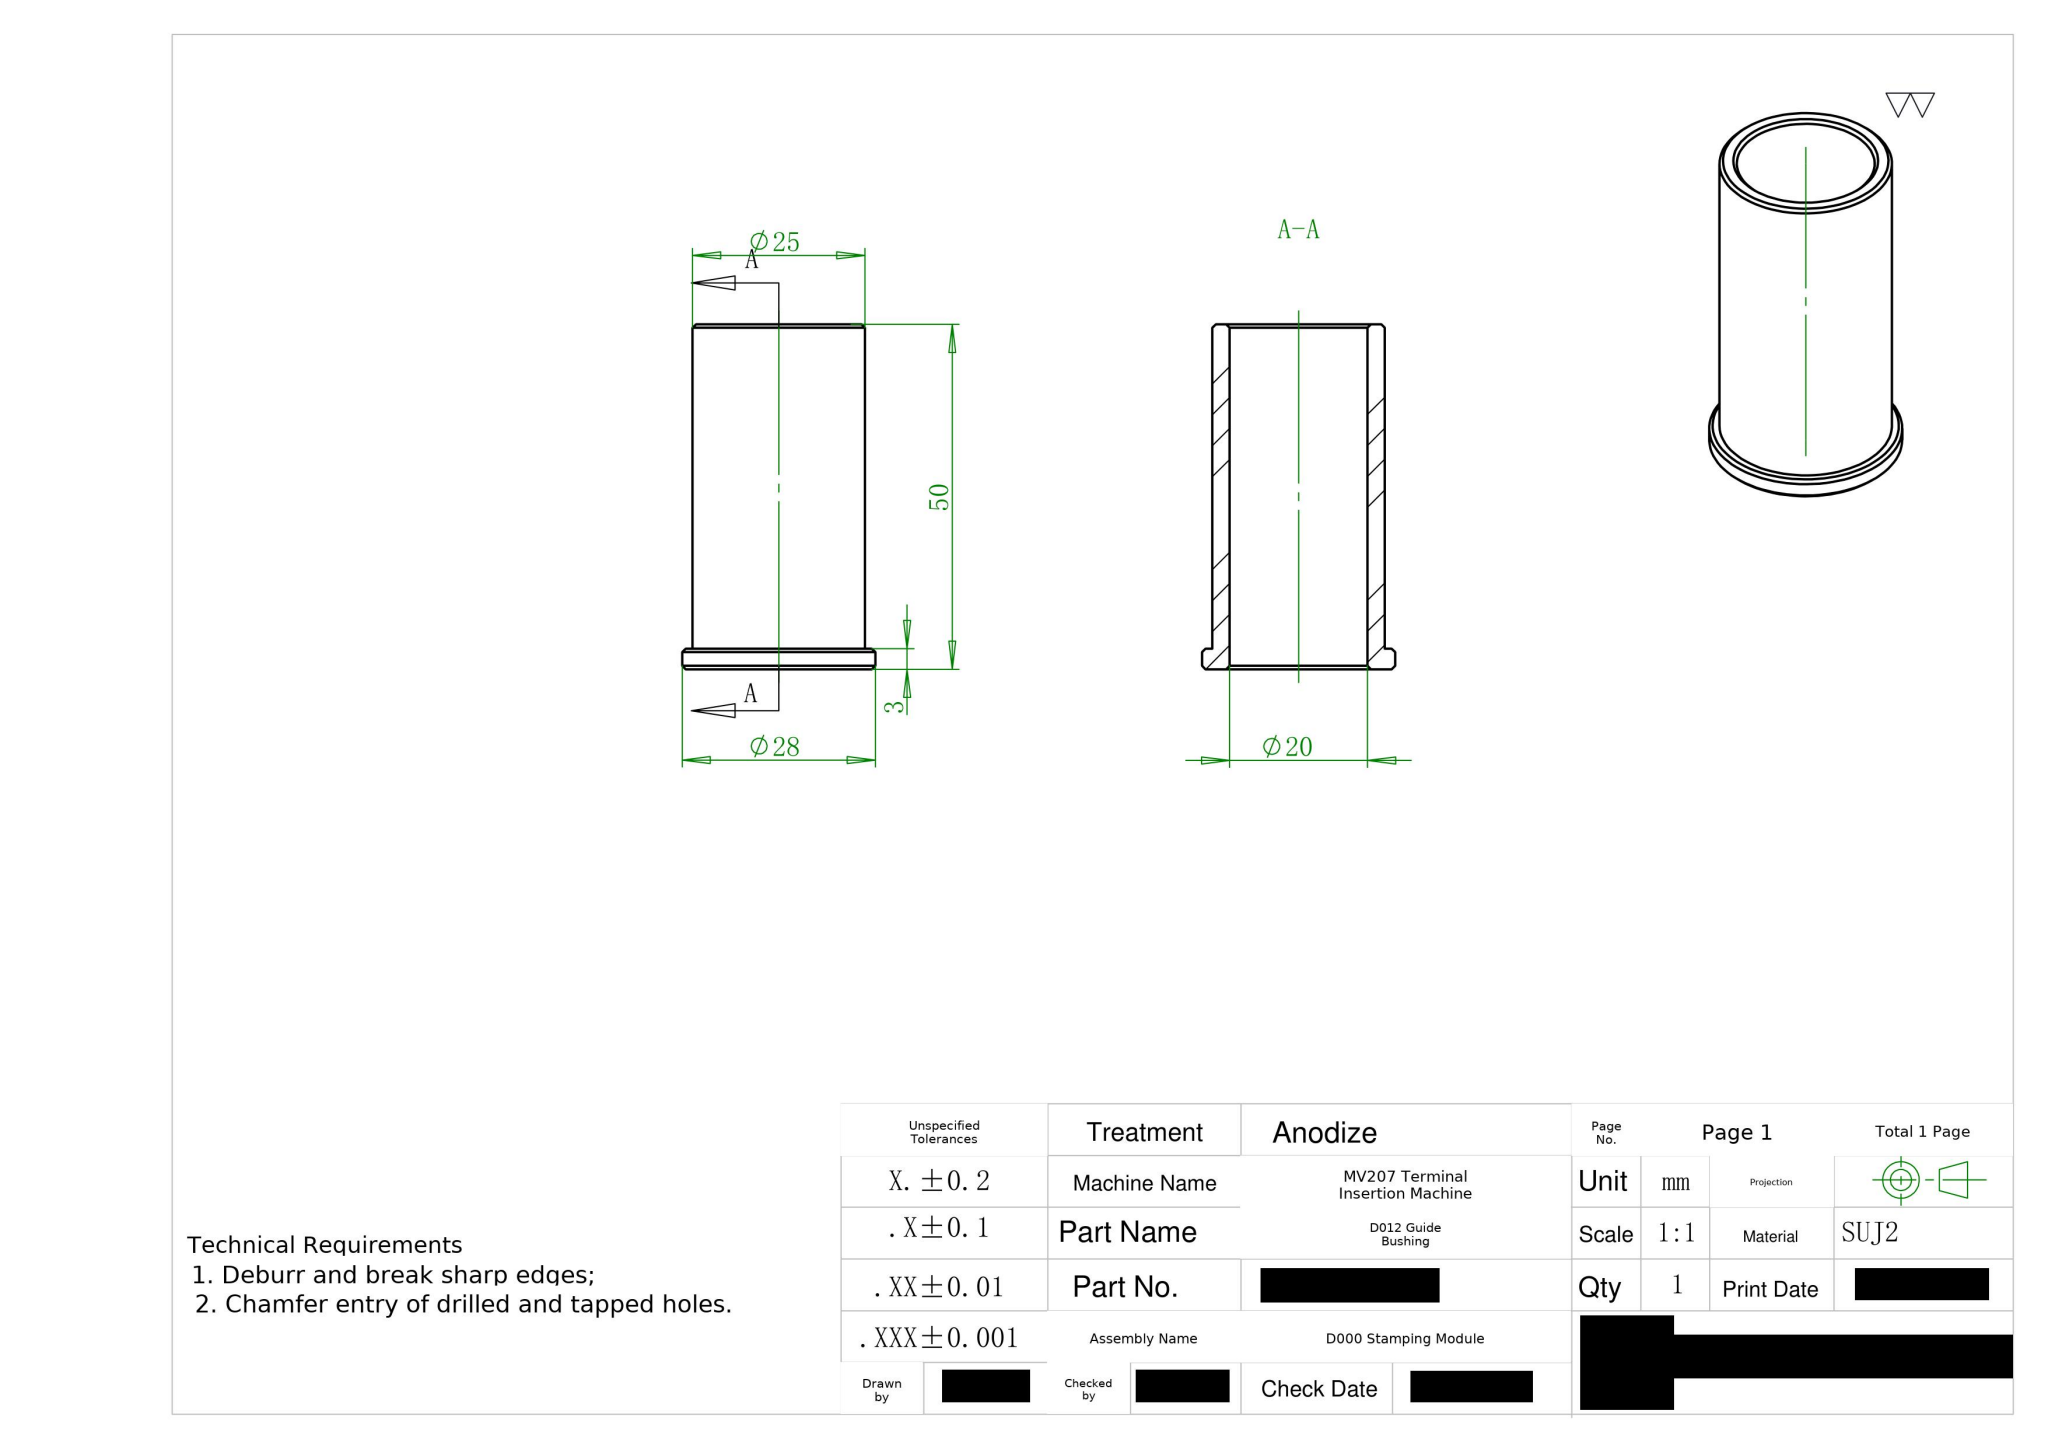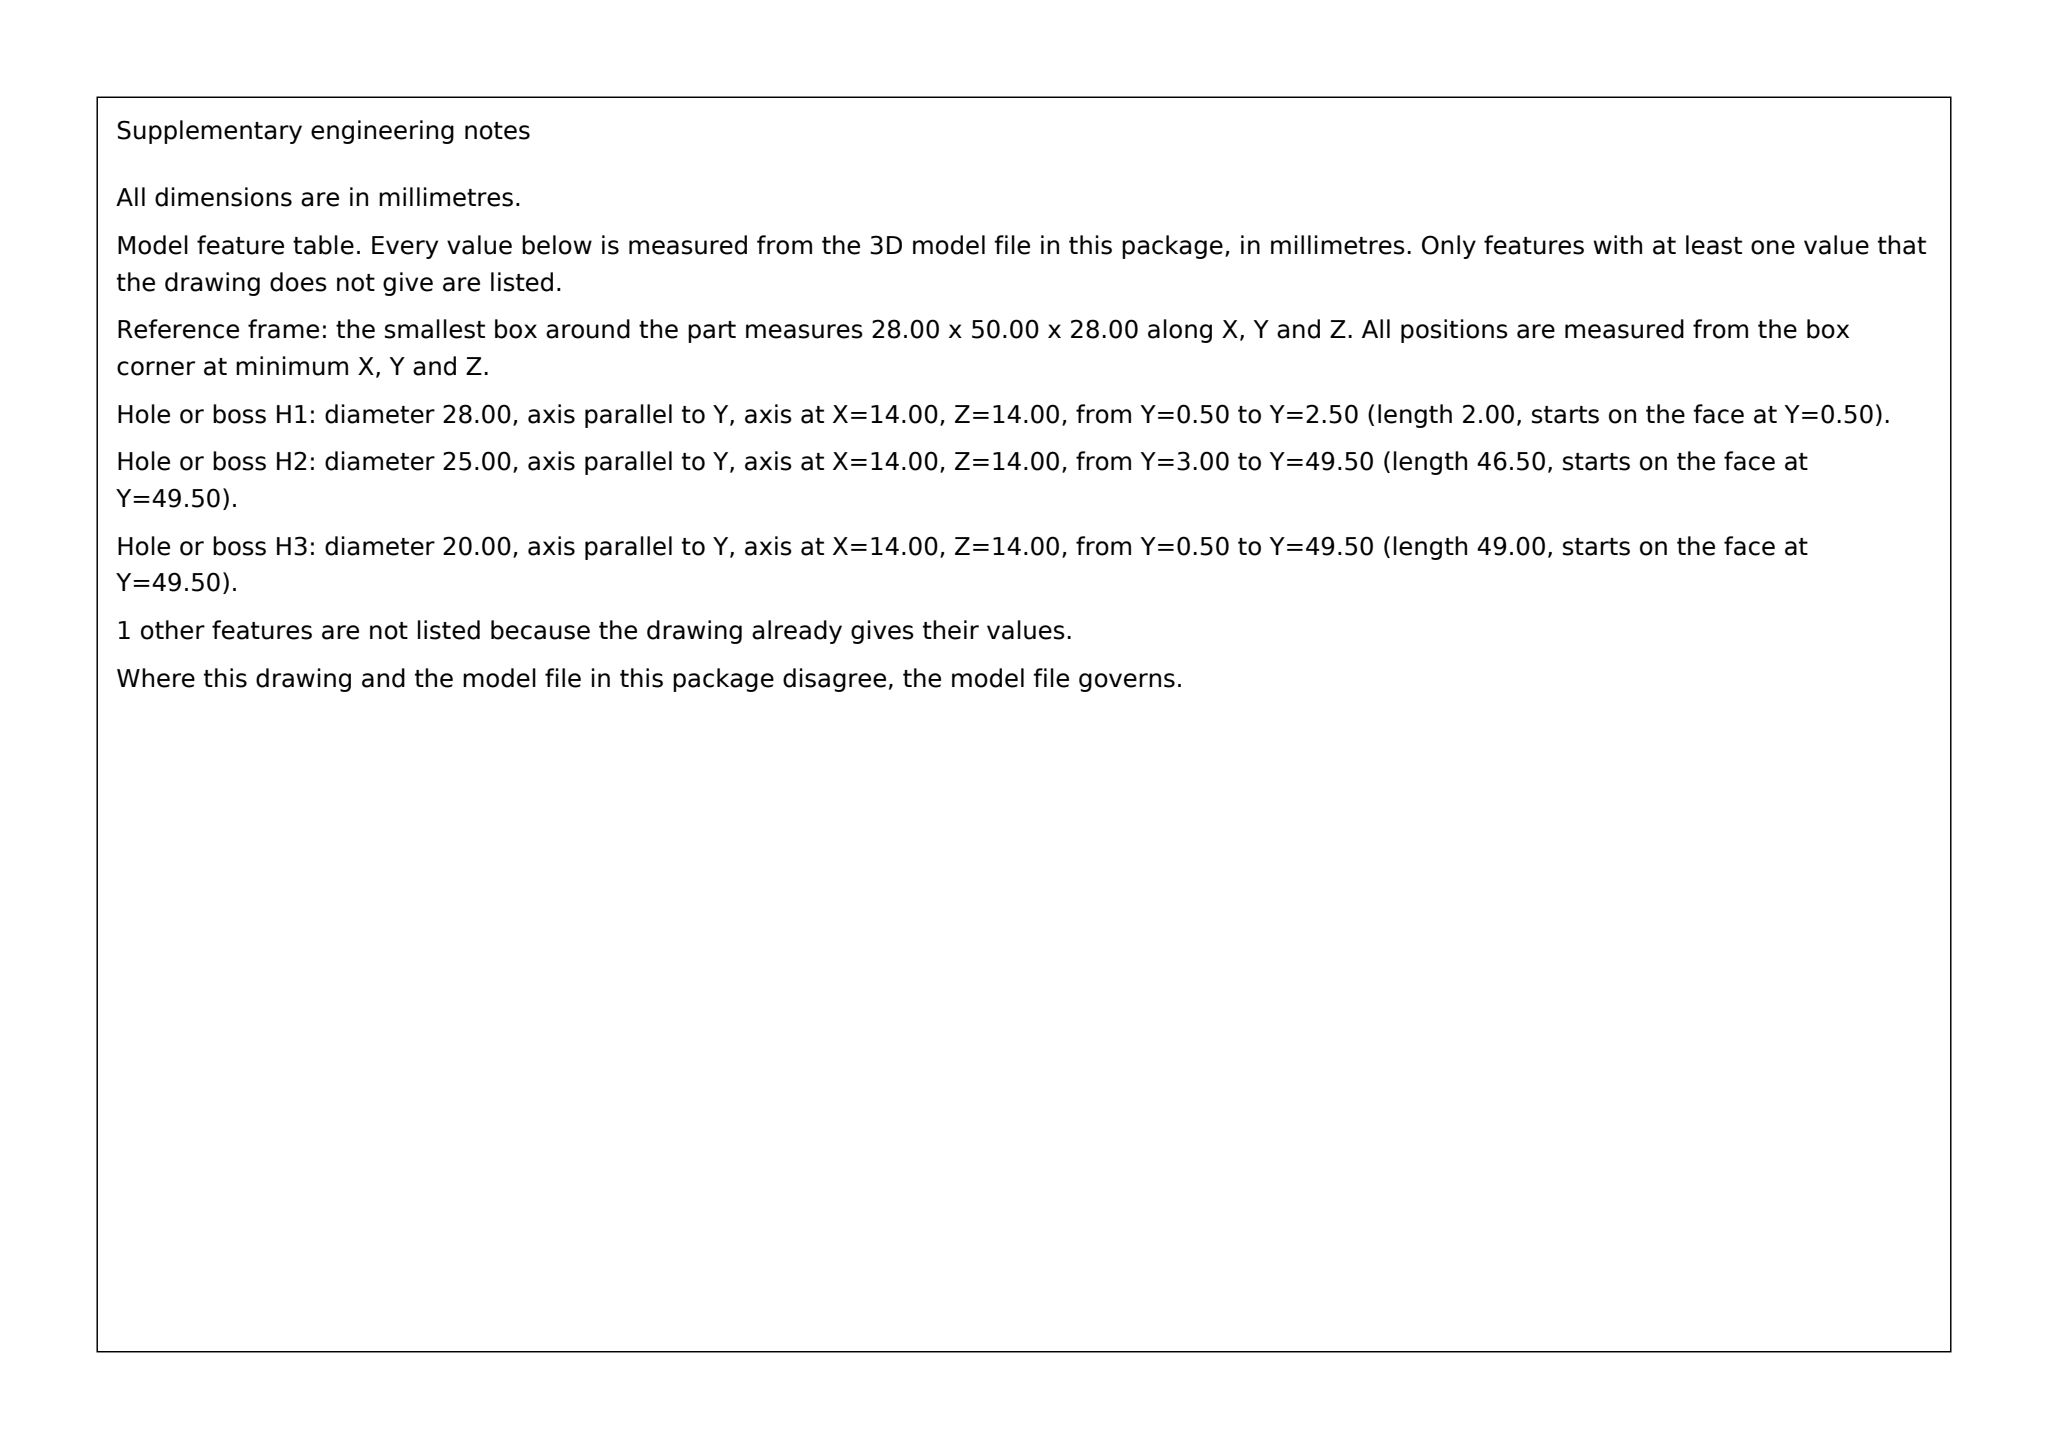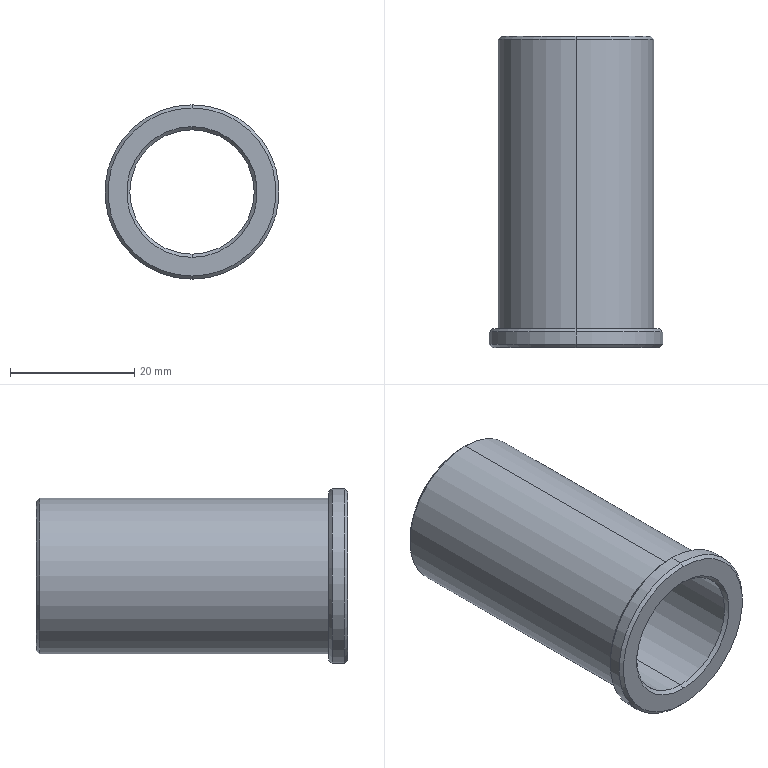Part | SolidWorks | mm | material SUJ2 | 1 solid | 19 faces | box 28 x 50 x 28 mm | volume 9163 mm3 | cone 10 | cylinder 6 | plane 3 | commonest cylinder face diameters 20 x2 25 x2 28 x2
build123d program:
from build123d import *

# Parameters (mm, degrees)
SKETCH1_R           = 14
BOSS_EXTRUDE1_DEPTH = 3
SKETCH2_R           = 12.5
BOSS_EXTRUDE2_DEPTH = 47
SKETCH3_R           = 10
CUT_EXTRUDE1_DEPTH  = 54.777
CHAMFER1_SIZE       = 0.5
CHAMFER2_SIZE       = 0.5


with BuildPart() as part:
    # Sketch1 → Boss-Extrude1 (new body)
    with BuildSketch(Plane(origin=(0, 0, 0), x_dir=(1, 0, 0), z_dir=(0, 1, 0))):
        with Locations(Location((0, 0, 0), (0, 0, 270))):
            Circle(SKETCH1_R)
    extrude(amount=BOSS_EXTRUDE1_DEPTH)

    # Sketch2 → Boss-Extrude2 (add)
    with BuildSketch(Plane(origin=(0, 3, 0), x_dir=(1, 0, 0), z_dir=(0, 1, 0))):
        with Locations(Location((0, 0, 0), (0, 0, 270))):
            Circle(SKETCH2_R)
    extrude(amount=BOSS_EXTRUDE2_DEPTH)

    # Sketch3 → Cut-Extrude1 (cut, through all)
    with BuildSketch(Plane.XZ):
        with Locations(Location((0, 0, 0), (0, 0, 270))):
            Circle(SKETCH3_R)
    extrude(amount=-CUT_EXTRUDE1_DEPTH, mode=Mode.SUBTRACT)

    # Chamfer1
    chamfer1_edges = [part.edges().sort_by_distance(p)[0] for p in [
        (0, 0, -14),
        (0, 3, -14),
    ]]
    chamfer(chamfer1_edges, length=CHAMFER1_SIZE)

    # Chamfer2
    chamfer2_edges = [part.edges().sort_by_distance(p)[0] for p in [
        (0, 50, 10),
        (0, 0, 10),
        (0, 50, -12.5),
    ]]
    chamfer(chamfer2_edges, length=CHAMFER2_SIZE)


solid = part.part
STEP:
#1=CARTESIAN_POINT('',(0.,0.5,10.));
#2=VERTEX_POINT('',#1);
#3=CARTESIAN_POINT('',(0.,0.5,-10.));
#4=VERTEX_POINT('',#3);
#5=CARTESIAN_POINT('',(0.,0.5,0.));
#6=DIRECTION('',(0.,-1.,0.));
#7=DIRECTION('',(0.,0.,1.));
#8=AXIS2_PLACEMENT_3D('',#5,#6,#7);
#9=CIRCLE('',#8,10.);
#10=EDGE_CURVE('',#2,#4,#9,.T.);
#11=ORIENTED_EDGE('',*,*,#10,.F.);
#12=CARTESIAN_POINT('',(0.,0.,10.5));
#13=VERTEX_POINT('',#12);
#14=CARTESIAN_POINT('',(0.,0.5,10.));
#15=DIRECTION('',(0.,-0.7071,0.7071));
#16=VECTOR('',#15,1000.);
#17=LINE('',#14,#16);
#18=EDGE_CURVE('',#2,#13,#17,.T.);
#19=ORIENTED_EDGE('',*,*,#18,.T.);
#20=CARTESIAN_POINT('',(0.,0.,-10.5));
#21=VERTEX_POINT('',#20);
#22=CARTESIAN_POINT('',(0.,0.,0.));
#23=DIRECTION('',(0.,1.,0.));
#24=DIRECTION('',(0.,0.,1.));
#25=AXIS2_PLACEMENT_3D('',#22,#23,#24);
#26=CIRCLE('',#25,10.5);
#27=EDGE_CURVE('',#21,#13,#26,.T.);
#28=ORIENTED_EDGE('',*,*,#27,.F.);
#29=CARTESIAN_POINT('',(0.,0.5,-10.));
#30=DIRECTION('',(0.,-0.7071,-0.7071));
#31=VECTOR('',#30,1000.);
#32=LINE('',#29,#31);
#33=EDGE_CURVE('',#4,#21,#32,.T.);
#34=ORIENTED_EDGE('',*,*,#33,.F.);
#35=EDGE_LOOP('',(#11,#19,#28,#34));
#36=FACE_OUTER_BOUND('',#35,.T.);
#37=CARTESIAN_POINT('',(0.,0.5,0.));
#38=DIRECTION('',(0.,-1.,0.));
#39=DIRECTION('',(0.,0.,-1.));
#40=AXIS2_PLACEMENT_3D('',#37,#38,#39);
#41=CONICAL_SURFACE('',#40,10.,0.7854);
#42=ADVANCED_FACE('',(#36),#41,.F.);
#43=CARTESIAN_POINT('',(0.,49.5,-10.));
#44=VERTEX_POINT('',#43);
#45=CARTESIAN_POINT('',(0.,49.5,10.));
#46=VERTEX_POINT('',#45);
#47=CARTESIAN_POINT('',(0.,49.5,0.));
#48=DIRECTION('',(0.,1.,0.));
#49=DIRECTION('',(0.,0.,1.));
#50=AXIS2_PLACEMENT_3D('',#47,#48,#49);
#51=CIRCLE('',#50,10.);
#52=EDGE_CURVE('',#44,#46,#51,.T.);
#53=ORIENTED_EDGE('',*,*,#52,.F.);
#54=CARTESIAN_POINT('',(0.,50.,-10.5));
#55=VERTEX_POINT('',#54);
#56=CARTESIAN_POINT('',(0.,50.,-10.5));
#57=DIRECTION('',(0.,0.7071,-0.7071));
#58=VECTOR('',#57,1000.);
#59=LINE('',#56,#58);
#60=EDGE_CURVE('',#44,#55,#59,.T.);
#61=ORIENTED_EDGE('',*,*,#60,.T.);
#62=CARTESIAN_POINT('',(0.,50.,10.5));
#63=VERTEX_POINT('',#62);
#64=CARTESIAN_POINT('',(0.,50.,0.));
#65=DIRECTION('',(0.,-1.,0.));
#66=DIRECTION('',(0.,0.,1.));
#67=AXIS2_PLACEMENT_3D('',#64,#65,#66);
#68=CIRCLE('',#67,10.5);
#69=EDGE_CURVE('',#63,#55,#68,.T.);
#70=ORIENTED_EDGE('',*,*,#69,.F.);
#71=CARTESIAN_POINT('',(0.,50.,10.5));
#72=DIRECTION('',(0.,0.7071,0.7071));
#73=VECTOR('',#72,1000.);
#74=LINE('',#71,#73);
#75=EDGE_CURVE('',#46,#63,#74,.T.);
#76=ORIENTED_EDGE('',*,*,#75,.F.);
#77=EDGE_LOOP('',(#53,#61,#70,#76));
#78=FACE_OUTER_BOUND('',#77,.T.);
#79=CARTESIAN_POINT('',(0.,50.,0.));
#80=DIRECTION('',(0.,1.,0.));
#81=DIRECTION('',(0.,0.,1.));
#82=AXIS2_PLACEMENT_3D('',#79,#80,#81);
#83=CONICAL_SURFACE('',#82,10.5,0.7854);
#84=ADVANCED_FACE('',(#78),#83,.F.);
#85=CARTESIAN_POINT('',(0.,50.,12.));
#86=VERTEX_POINT('',#85);
#87=CARTESIAN_POINT('',(0.,50.,-12.));
#88=VERTEX_POINT('',#87);
#89=CARTESIAN_POINT('',(0.,50.,0.));
#90=DIRECTION('',(0.,1.,0.));
#91=DIRECTION('',(0.,0.,1.));
#92=AXIS2_PLACEMENT_3D('',#89,#90,#91);
#93=CIRCLE('',#92,12.);
#94=EDGE_CURVE('',#86,#88,#93,.T.);
#95=ORIENTED_EDGE('',*,*,#94,.F.);
#96=CARTESIAN_POINT('',(0.,49.5,12.5));
#97=VERTEX_POINT('',#96);
#98=CARTESIAN_POINT('',(0.,50.,12.));
#99=DIRECTION('',(0.,-0.7071,0.7071));
#100=VECTOR('',#99,1000.);
#101=LINE('',#98,#100);
#102=EDGE_CURVE('',#86,#97,#101,.T.);
#103=ORIENTED_EDGE('',*,*,#102,.T.);
#104=CARTESIAN_POINT('',(0.,49.5,-12.5));
#105=VERTEX_POINT('',#104);
#106=CARTESIAN_POINT('',(0.,49.5,0.));
#107=DIRECTION('',(0.,-1.,0.));
#108=DIRECTION('',(0.,0.,1.));
#109=AXIS2_PLACEMENT_3D('',#106,#107,#108);
#110=CIRCLE('',#109,12.5);
#111=EDGE_CURVE('',#105,#97,#110,.T.);
#112=ORIENTED_EDGE('',*,*,#111,.F.);
#113=CARTESIAN_POINT('',(0.,50.,-12.));
#114=DIRECTION('',(0.,-0.7071,-0.7071));
#115=VECTOR('',#114,1000.);
#116=LINE('',#113,#115);
#117=EDGE_CURVE('',#88,#105,#116,.T.);
#118=ORIENTED_EDGE('',*,*,#117,.F.);
#119=EDGE_LOOP('',(#95,#103,#112,#118));
#120=FACE_OUTER_BOUND('',#119,.T.);
#121=CARTESIAN_POINT('',(0.,50.,0.));
#122=DIRECTION('',(0.,-1.,0.));
#123=DIRECTION('',(0.,0.,-1.));
#124=AXIS2_PLACEMENT_3D('',#121,#122,#123);
#125=CONICAL_SURFACE('',#124,12.,0.7854);
#126=ADVANCED_FACE('',(#120),#125,.T.);
#127=CARTESIAN_POINT('',(0.,3.,13.5));
#128=VERTEX_POINT('',#127);
#129=CARTESIAN_POINT('',(0.,3.,-13.5));
#130=VERTEX_POINT('',#129);
#131=CARTESIAN_POINT('',(0.,3.,0.));
#132=DIRECTION('',(0.,1.,0.));
#133=DIRECTION('',(0.,0.,1.));
#134=AXIS2_PLACEMENT_3D('',#131,#132,#133);
#135=CIRCLE('',#134,13.5);
#136=EDGE_CURVE('',#128,#130,#135,.T.);
#137=ORIENTED_EDGE('',*,*,#136,.F.);
#138=CARTESIAN_POINT('',(0.,2.5,14.));
#139=VERTEX_POINT('',#138);
#140=CARTESIAN_POINT('',(0.,3.,13.5));
#141=DIRECTION('',(0.,-0.7071,0.7071));
#142=VECTOR('',#141,1000.);
#143=LINE('',#140,#142);
#144=EDGE_CURVE('',#128,#139,#143,.T.);
#145=ORIENTED_EDGE('',*,*,#144,.T.);
#146=CARTESIAN_POINT('',(0.,2.5,-14.));
#147=VERTEX_POINT('',#146);
#148=CARTESIAN_POINT('',(0.,2.5,0.));
#149=DIRECTION('',(0.,-1.,0.));
#150=DIRECTION('',(0.,0.,1.));
#151=AXIS2_PLACEMENT_3D('',#148,#149,#150);
#152=CIRCLE('',#151,14.);
#153=EDGE_CURVE('',#147,#139,#152,.T.);
#154=ORIENTED_EDGE('',*,*,#153,.F.);
#155=CARTESIAN_POINT('',(0.,3.,-13.5));
#156=DIRECTION('',(0.,-0.7071,-0.7071));
#157=VECTOR('',#156,1000.);
#158=LINE('',#155,#157);
#159=EDGE_CURVE('',#130,#147,#158,.T.);
#160=ORIENTED_EDGE('',*,*,#159,.F.);
#161=EDGE_LOOP('',(#137,#145,#154,#160));
#162=FACE_OUTER_BOUND('',#161,.T.);
#163=CARTESIAN_POINT('',(0.,3.,0.));
#164=DIRECTION('',(0.,-1.,0.));
#165=DIRECTION('',(0.,0.,-1.));
#166=AXIS2_PLACEMENT_3D('',#163,#164,#165);
#167=CONICAL_SURFACE('',#166,13.5,0.7854);
#168=ADVANCED_FACE('',(#162),#167,.T.);
#169=CARTESIAN_POINT('',(0.,0.,-13.5));
#170=VERTEX_POINT('',#169);
#171=CARTESIAN_POINT('',(0.,0.,13.5));
#172=VERTEX_POINT('',#171);
#173=CARTESIAN_POINT('',(0.,0.,0.));
#174=DIRECTION('',(0.,-1.,0.));
#175=DIRECTION('',(0.,0.,1.));
#176=AXIS2_PLACEMENT_3D('',#173,#174,#175);
#177=CIRCLE('',#176,13.5);
#178=EDGE_CURVE('',#170,#172,#177,.T.);
#179=ORIENTED_EDGE('',*,*,#178,.F.);
#180=CARTESIAN_POINT('',(0.,0.5,-14.));
#181=VERTEX_POINT('',#180);
#182=CARTESIAN_POINT('',(0.,0.5,-14.));
#183=DIRECTION('',(0.,0.7071,-0.7071));
#184=VECTOR('',#183,1000.);
#185=LINE('',#182,#184);
#186=EDGE_CURVE('',#170,#181,#185,.T.);
#187=ORIENTED_EDGE('',*,*,#186,.T.);
#188=CARTESIAN_POINT('',(0.,0.5,14.));
#189=VERTEX_POINT('',#188);
#190=CARTESIAN_POINT('',(0.,0.5,0.));
#191=DIRECTION('',(0.,1.,0.));
#192=DIRECTION('',(0.,0.,1.));
#193=AXIS2_PLACEMENT_3D('',#190,#191,#192);
#194=CIRCLE('',#193,14.);
#195=EDGE_CURVE('',#189,#181,#194,.T.);
#196=ORIENTED_EDGE('',*,*,#195,.F.);
#197=CARTESIAN_POINT('',(0.,0.5,14.));
#198=DIRECTION('',(0.,0.7071,0.7071));
#199=VECTOR('',#198,1000.);
#200=LINE('',#197,#199);
#201=EDGE_CURVE('',#172,#189,#200,.T.);
#202=ORIENTED_EDGE('',*,*,#201,.F.);
#203=EDGE_LOOP('',(#179,#187,#196,#202));
#204=FACE_OUTER_BOUND('',#203,.T.);
#205=CARTESIAN_POINT('',(0.,0.5,0.));
#206=DIRECTION('',(0.,1.,0.));
#207=DIRECTION('',(0.,0.,1.));
#208=AXIS2_PLACEMENT_3D('',#205,#206,#207);
#209=CONICAL_SURFACE('',#208,14.,0.7854);
#210=ADVANCED_FACE('',(#204),#209,.T.);
#211=ORIENTED_EDGE('',*,*,#52,.T.);
#212=CARTESIAN_POINT('',(0.,50.,10.));
#213=DIRECTION('',(0.,-1.,0.));
#214=VECTOR('',#213,1000.);
#215=LINE('',#212,#214);
#216=EDGE_CURVE('',#46,#2,#215,.T.);
#217=ORIENTED_EDGE('',*,*,#216,.T.);
#218=ORIENTED_EDGE('',*,*,#10,.T.);
#219=CARTESIAN_POINT('',(0.,50.,-10.));
#220=DIRECTION('',(0.,-1.,0.));
#221=VECTOR('',#220,1000.);
#222=LINE('',#219,#221);
#223=EDGE_CURVE('',#44,#4,#222,.T.);
#224=ORIENTED_EDGE('',*,*,#223,.F.);
#225=EDGE_LOOP('',(#211,#217,#218,#224));
#226=FACE_OUTER_BOUND('',#225,.T.);
#227=CARTESIAN_POINT('',(0.,50.,0.));
#228=DIRECTION('',(0.,-1.,0.));
#229=DIRECTION('',(0.,0.,-1.));
#230=AXIS2_PLACEMENT_3D('',#227,#228,#229);
#231=CYLINDRICAL_SURFACE('',#230,10.);
#232=ADVANCED_FACE('',(#226),#231,.F.);
#233=ORIENTED_EDGE('',*,*,#111,.T.);
#234=CARTESIAN_POINT('',(0.,3.,12.5));
#235=VERTEX_POINT('',#234);
#236=CARTESIAN_POINT('',(0.,50.,12.5));
#237=DIRECTION('',(0.,-1.,0.));
#238=VECTOR('',#237,1000.);
#239=LINE('',#236,#238);
#240=EDGE_CURVE('',#97,#235,#239,.T.);
#241=ORIENTED_EDGE('',*,*,#240,.T.);
#242=CARTESIAN_POINT('',(0.,3.,-12.5));
#243=VERTEX_POINT('',#242);
#244=CARTESIAN_POINT('',(0.,3.,0.));
#245=DIRECTION('',(0.,1.,0.));
#246=DIRECTION('',(0.,0.,1.));
#247=AXIS2_PLACEMENT_3D('',#244,#245,#246);
#248=CIRCLE('',#247,12.5);
#249=EDGE_CURVE('',#235,#243,#248,.T.);
#250=ORIENTED_EDGE('',*,*,#249,.T.);
#251=CARTESIAN_POINT('',(0.,50.,-12.5));
#252=DIRECTION('',(0.,-1.,0.));
#253=VECTOR('',#252,1000.);
#254=LINE('',#251,#253);
#255=EDGE_CURVE('',#105,#243,#254,.T.);
#256=ORIENTED_EDGE('',*,*,#255,.F.);
#257=EDGE_LOOP('',(#233,#241,#250,#256));
#258=FACE_OUTER_BOUND('',#257,.T.);
#259=CARTESIAN_POINT('',(0.,50.,0.));
#260=DIRECTION('',(0.,-1.,0.));
#261=DIRECTION('',(0.,0.,-1.));
#262=AXIS2_PLACEMENT_3D('',#259,#260,#261);
#263=CYLINDRICAL_SURFACE('',#262,12.5);
#264=ADVANCED_FACE('',(#258),#263,.T.);
#265=ORIENTED_EDGE('',*,*,#153,.T.);
#266=CARTESIAN_POINT('',(0.,3.,14.));
#267=DIRECTION('',(0.,-1.,0.));
#268=VECTOR('',#267,1000.);
#269=LINE('',#266,#268);
#270=EDGE_CURVE('',#139,#189,#269,.T.);
#271=ORIENTED_EDGE('',*,*,#270,.T.);
#272=ORIENTED_EDGE('',*,*,#195,.T.);
#273=CARTESIAN_POINT('',(0.,3.,-14.));
#274=DIRECTION('',(0.,-1.,0.));
#275=VECTOR('',#274,1000.);
#276=LINE('',#273,#275);
#277=EDGE_CURVE('',#147,#181,#276,.T.);
#278=ORIENTED_EDGE('',*,*,#277,.F.);
#279=EDGE_LOOP('',(#265,#271,#272,#278));
#280=FACE_OUTER_BOUND('',#279,.T.);
#281=CARTESIAN_POINT('',(0.,3.,0.));
#282=DIRECTION('',(0.,-1.,0.));
#283=DIRECTION('',(0.,0.,-1.));
#284=AXIS2_PLACEMENT_3D('',#281,#282,#283);
#285=CYLINDRICAL_SURFACE('',#284,14.);
#286=ADVANCED_FACE('',(#280),#285,.T.);
#287=CARTESIAN_POINT('',(0.,3.,0.));
#288=DIRECTION('',(0.,1.,0.));
#289=DIRECTION('',(0.,0.,1.));
#290=AXIS2_PLACEMENT_3D('',#287,#288,#289);
#291=CIRCLE('',#290,13.5);
#292=EDGE_CURVE('',#130,#128,#291,.T.);
#293=ORIENTED_EDGE('',*,*,#292,.T.);
#294=ORIENTED_EDGE('',*,*,#136,.T.);
#295=EDGE_LOOP('',(#293,#294));
#296=FACE_OUTER_BOUND('',#295,.T.);
#297=CARTESIAN_POINT('',(0.,3.,0.));
#298=DIRECTION('',(0.,1.,0.));
#299=DIRECTION('',(0.,0.,1.));
#300=AXIS2_PLACEMENT_3D('',#297,#298,#299);
#301=CIRCLE('',#300,12.5);
#302=EDGE_CURVE('',#243,#235,#301,.T.);
#303=ORIENTED_EDGE('',*,*,#302,.F.);
#304=ORIENTED_EDGE('',*,*,#249,.F.);
#305=EDGE_LOOP('',(#303,#304));
#306=FACE_BOUND('',#305,.T.);
#307=CARTESIAN_POINT('',(0.,3.,0.));
#308=DIRECTION('',(0.,1.,0.));
#309=DIRECTION('',(0.,0.,1.));
#310=AXIS2_PLACEMENT_3D('',#307,#308,#309);
#311=PLANE('',#310);
#312=ADVANCED_FACE('',(#296,#306),#311,.T.);
#313=ORIENTED_EDGE('',*,*,#270,.F.);
#314=CARTESIAN_POINT('',(0.,2.5,0.));
#315=DIRECTION('',(0.,-1.,0.));
#316=DIRECTION('',(0.,0.,1.));
#317=AXIS2_PLACEMENT_3D('',#314,#315,#316);
#318=CIRCLE('',#317,14.);
#319=EDGE_CURVE('',#139,#147,#318,.T.);
#320=ORIENTED_EDGE('',*,*,#319,.T.);
#321=ORIENTED_EDGE('',*,*,#277,.T.);
#322=CARTESIAN_POINT('',(0.,0.5,0.));
#323=DIRECTION('',(0.,1.,0.));
#324=DIRECTION('',(0.,0.,1.));
#325=AXIS2_PLACEMENT_3D('',#322,#323,#324);
#326=CIRCLE('',#325,14.);
#327=EDGE_CURVE('',#181,#189,#326,.T.);
#328=ORIENTED_EDGE('',*,*,#327,.T.);
#329=EDGE_LOOP('',(#313,#320,#321,#328));
#330=FACE_OUTER_BOUND('',#329,.T.);
#331=CARTESIAN_POINT('',(0.,3.,0.));
#332=DIRECTION('',(0.,-1.,0.));
#333=DIRECTION('',(0.,0.,-1.));
#334=AXIS2_PLACEMENT_3D('',#331,#332,#333);
#335=CYLINDRICAL_SURFACE('',#334,14.);
#336=ADVANCED_FACE('',(#330),#335,.T.);
#337=ORIENTED_EDGE('',*,*,#27,.T.);
#338=CARTESIAN_POINT('',(0.,0.,0.));
#339=DIRECTION('',(0.,1.,0.));
#340=DIRECTION('',(0.,0.,1.));
#341=AXIS2_PLACEMENT_3D('',#338,#339,#340);
#342=CIRCLE('',#341,10.5);
#343=EDGE_CURVE('',#13,#21,#342,.T.);
#344=ORIENTED_EDGE('',*,*,#343,.T.);
#345=EDGE_LOOP('',(#337,#344));
#346=FACE_BOUND('',#345,.T.);
#347=CARTESIAN_POINT('',(0.,0.,0.));
#348=DIRECTION('',(0.,-1.,0.));
#349=DIRECTION('',(0.,0.,1.));
#350=AXIS2_PLACEMENT_3D('',#347,#348,#349);
#351=CIRCLE('',#350,13.5);
#352=EDGE_CURVE('',#172,#170,#351,.T.);
#353=ORIENTED_EDGE('',*,*,#352,.T.);
#354=ORIENTED_EDGE('',*,*,#178,.T.);
#355=EDGE_LOOP('',(#353,#354));
#356=FACE_OUTER_BOUND('',#355,.T.);
#357=CARTESIAN_POINT('',(0.,0.,0.));
#358=DIRECTION('',(0.,1.,0.));
#359=DIRECTION('',(0.,0.,1.));
#360=AXIS2_PLACEMENT_3D('',#357,#358,#359);
#361=PLANE('',#360);
#362=ADVANCED_FACE('',(#346,#356),#361,.F.);
#363=ORIENTED_EDGE('',*,*,#240,.F.);
#364=CARTESIAN_POINT('',(0.,49.5,0.));
#365=DIRECTION('',(0.,-1.,0.));
#366=DIRECTION('',(0.,0.,1.));
#367=AXIS2_PLACEMENT_3D('',#364,#365,#366);
#368=CIRCLE('',#367,12.5);
#369=EDGE_CURVE('',#97,#105,#368,.T.);
#370=ORIENTED_EDGE('',*,*,#369,.T.);
#371=ORIENTED_EDGE('',*,*,#255,.T.);
#372=ORIENTED_EDGE('',*,*,#302,.T.);
#373=EDGE_LOOP('',(#363,#370,#371,#372));
#374=FACE_OUTER_BOUND('',#373,.T.);
#375=CARTESIAN_POINT('',(0.,50.,0.));
#376=DIRECTION('',(0.,-1.,0.));
#377=DIRECTION('',(0.,0.,-1.));
#378=AXIS2_PLACEMENT_3D('',#375,#376,#377);
#379=CYLINDRICAL_SURFACE('',#378,12.5);
#380=ADVANCED_FACE('',(#374),#379,.T.);
#381=CARTESIAN_POINT('',(0.,50.,0.));
#382=DIRECTION('',(0.,1.,0.));
#383=DIRECTION('',(0.,0.,1.));
#384=AXIS2_PLACEMENT_3D('',#381,#382,#383);
#385=CIRCLE('',#384,12.);
#386=EDGE_CURVE('',#88,#86,#385,.T.);
#387=ORIENTED_EDGE('',*,*,#386,.T.);
#388=ORIENTED_EDGE('',*,*,#94,.T.);
#389=EDGE_LOOP('',(#387,#388));
#390=FACE_OUTER_BOUND('',#389,.T.);
#391=ORIENTED_EDGE('',*,*,#69,.T.);
#392=CARTESIAN_POINT('',(0.,50.,0.));
#393=DIRECTION('',(0.,-1.,0.));
#394=DIRECTION('',(0.,0.,1.));
#395=AXIS2_PLACEMENT_3D('',#392,#393,#394);
#396=CIRCLE('',#395,10.5);
#397=EDGE_CURVE('',#55,#63,#396,.T.);
#398=ORIENTED_EDGE('',*,*,#397,.T.);
#399=EDGE_LOOP('',(#391,#398));
#400=FACE_BOUND('',#399,.T.);
#401=CARTESIAN_POINT('',(0.,50.,0.));
#402=DIRECTION('',(0.,1.,0.));
#403=DIRECTION('',(0.,0.,1.));
#404=AXIS2_PLACEMENT_3D('',#401,#402,#403);
#405=PLANE('',#404);
#406=ADVANCED_FACE('',(#390,#400),#405,.T.);
#407=ORIENTED_EDGE('',*,*,#216,.F.);
#408=CARTESIAN_POINT('',(0.,49.5,0.));
#409=DIRECTION('',(0.,1.,0.));
#410=DIRECTION('',(0.,0.,1.));
#411=AXIS2_PLACEMENT_3D('',#408,#409,#410);
#412=CIRCLE('',#411,10.);
#413=EDGE_CURVE('',#46,#44,#412,.T.);
#414=ORIENTED_EDGE('',*,*,#413,.T.);
#415=ORIENTED_EDGE('',*,*,#223,.T.);
#416=CARTESIAN_POINT('',(0.,0.5,0.));
#417=DIRECTION('',(0.,-1.,0.));
#418=DIRECTION('',(0.,0.,1.));
#419=AXIS2_PLACEMENT_3D('',#416,#417,#418);
#420=CIRCLE('',#419,10.);
#421=EDGE_CURVE('',#4,#2,#420,.T.);
#422=ORIENTED_EDGE('',*,*,#421,.T.);
#423=EDGE_LOOP('',(#407,#414,#415,#422));
#424=FACE_OUTER_BOUND('',#423,.T.);
#425=CARTESIAN_POINT('',(0.,50.,0.));
#426=DIRECTION('',(0.,-1.,0.));
#427=DIRECTION('',(0.,0.,-1.));
#428=AXIS2_PLACEMENT_3D('',#425,#426,#427);
#429=CYLINDRICAL_SURFACE('',#428,10.);
#430=ADVANCED_FACE('',(#424),#429,.F.);
#431=ORIENTED_EDGE('',*,*,#186,.F.);
#432=ORIENTED_EDGE('',*,*,#352,.F.);
#433=ORIENTED_EDGE('',*,*,#201,.T.);
#434=ORIENTED_EDGE('',*,*,#327,.F.);
#435=EDGE_LOOP('',(#431,#432,#433,#434));
#436=FACE_OUTER_BOUND('',#435,.T.);
#437=CARTESIAN_POINT('',(0.,0.5,0.));
#438=DIRECTION('',(0.,1.,0.));
#439=DIRECTION('',(0.,0.,1.));
#440=AXIS2_PLACEMENT_3D('',#437,#438,#439);
#441=CONICAL_SURFACE('',#440,14.,0.7854);
#442=ADVANCED_FACE('',(#436),#441,.T.);
#443=ORIENTED_EDGE('',*,*,#144,.F.);
#444=ORIENTED_EDGE('',*,*,#292,.F.);
#445=ORIENTED_EDGE('',*,*,#159,.T.);
#446=ORIENTED_EDGE('',*,*,#319,.F.);
#447=EDGE_LOOP('',(#443,#444,#445,#446));
#448=FACE_OUTER_BOUND('',#447,.T.);
#449=CARTESIAN_POINT('',(0.,3.,0.));
#450=DIRECTION('',(0.,-1.,0.));
#451=DIRECTION('',(0.,0.,-1.));
#452=AXIS2_PLACEMENT_3D('',#449,#450,#451);
#453=CONICAL_SURFACE('',#452,13.5,0.7854);
#454=ADVANCED_FACE('',(#448),#453,.T.);
#455=ORIENTED_EDGE('',*,*,#102,.F.);
#456=ORIENTED_EDGE('',*,*,#386,.F.);
#457=ORIENTED_EDGE('',*,*,#117,.T.);
#458=ORIENTED_EDGE('',*,*,#369,.F.);
#459=EDGE_LOOP('',(#455,#456,#457,#458));
#460=FACE_OUTER_BOUND('',#459,.T.);
#461=CARTESIAN_POINT('',(0.,50.,0.));
#462=DIRECTION('',(0.,-1.,0.));
#463=DIRECTION('',(0.,0.,-1.));
#464=AXIS2_PLACEMENT_3D('',#461,#462,#463);
#465=CONICAL_SURFACE('',#464,12.,0.7854);
#466=ADVANCED_FACE('',(#460),#465,.T.);
#467=ORIENTED_EDGE('',*,*,#60,.F.);
#468=ORIENTED_EDGE('',*,*,#413,.F.);
#469=ORIENTED_EDGE('',*,*,#75,.T.);
#470=ORIENTED_EDGE('',*,*,#397,.F.);
#471=EDGE_LOOP('',(#467,#468,#469,#470));
#472=FACE_OUTER_BOUND('',#471,.T.);
#473=CARTESIAN_POINT('',(0.,50.,0.));
#474=DIRECTION('',(0.,1.,0.));
#475=DIRECTION('',(0.,0.,1.));
#476=AXIS2_PLACEMENT_3D('',#473,#474,#475);
#477=CONICAL_SURFACE('',#476,10.5,0.7854);
#478=ADVANCED_FACE('',(#472),#477,.F.);
#479=ORIENTED_EDGE('',*,*,#18,.F.);
#480=ORIENTED_EDGE('',*,*,#421,.F.);
#481=ORIENTED_EDGE('',*,*,#33,.T.);
#482=ORIENTED_EDGE('',*,*,#343,.F.);
#483=EDGE_LOOP('',(#479,#480,#481,#482));
#484=FACE_OUTER_BOUND('',#483,.T.);
#485=CARTESIAN_POINT('',(0.,0.5,0.));
#486=DIRECTION('',(0.,-1.,0.));
#487=DIRECTION('',(0.,0.,-1.));
#488=AXIS2_PLACEMENT_3D('',#485,#486,#487);
#489=CONICAL_SURFACE('',#488,10.,0.7854);
#490=ADVANCED_FACE('',(#484),#489,.F.);
#491=CLOSED_SHELL('',(#42,#84,#126,#168,#210,#232,#264,#286,#312,#336,#362,#380,#406,#430,#442,#454,#466,#478,#490));
#492=MANIFOLD_SOLID_BREP('',#491);
#493=CARTESIAN_POINT('',(0.,0.,0.));
#494=DIRECTION('',(0.,0.,1.));
#495=DIRECTION('',(1.,0.,0.));
#496=AXIS2_PLACEMENT_3D('',#493,#494,#495);
#497=(LENGTH_UNIT()NAMED_UNIT(*)SI_UNIT(.MILLI.,.METRE.));
#498=UNCERTAINTY_MEASURE_WITH_UNIT(LENGTH_MEASURE(0.00001),#497,'','');
#499=(NAMED_UNIT(*)PLANE_ANGLE_UNIT()SI_UNIT($,.RADIAN.));
#500=(NAMED_UNIT(*)SI_UNIT($,.STERADIAN.)SOLID_ANGLE_UNIT());
#501=(GEOMETRIC_REPRESENTATION_CONTEXT(3)GLOBAL_UNCERTAINTY_ASSIGNED_CONTEXT((#498))GLOBAL_UNIT_ASSIGNED_CONTEXT((#497,#499,#500))REPRESENTATION_CONTEXT('',''));
#502=ADVANCED_BREP_SHAPE_REPRESENTATION('',(#492,#496),#501);